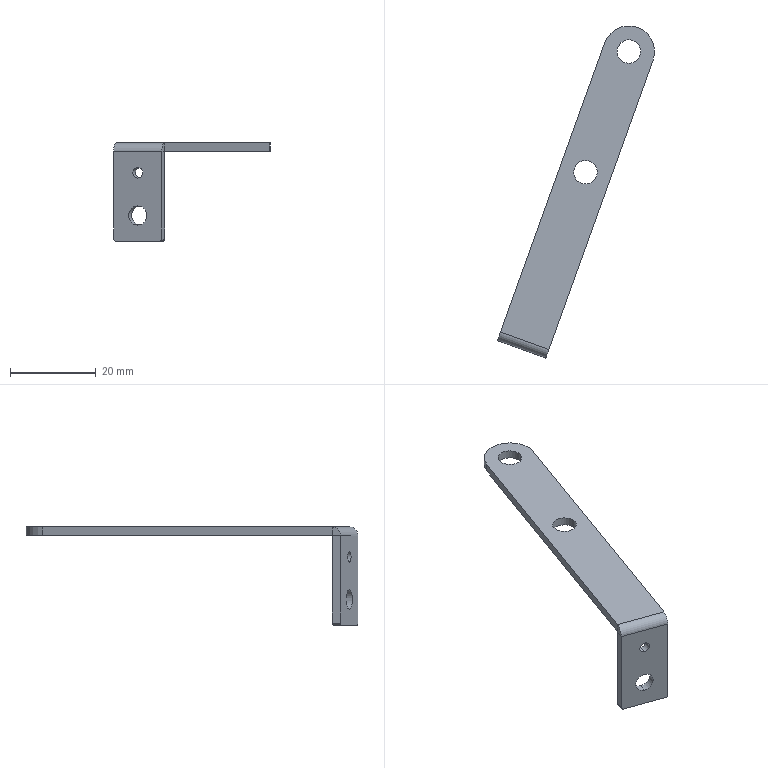Component | SolidWorks | CLS-MechanismAccessory4-1 | 1 solid | 25 faces | box 36.72 x 77.65 x 23 mm | volume 2245 mm3 | cylinder 14 | plane 11 | commonest cylinder face diameters 5.5 x4 2.5 x2 4.5 x2 12 x2 1 x2 4.2 x1 0.2 x1 | material 2.0 Galvanized Sheet Q235A
STEP:
#1=CARTESIAN_POINT('',(1.545,-2.454,-0.3445));
#2=VERTEX_POINT('',#1);
#3=CARTESIAN_POINT('',(1.545,-2.454,-0.4429));
#4=VERTEX_POINT('',#3);
#5=CARTESIAN_POINT('',(1.545,-2.454,-0.3937));
#6=DIRECTION('',(-0.3389,-0.9408,0.));
#7=DIRECTION('',(0.,-0.,-1.));
#8=AXIS2_PLACEMENT_3D('',#5,#6,#7);
#9=CIRCLE('',#8,0.04921);
#10=EDGE_CURVE('',#2,#4,#9,.T.);
#11=ORIENTED_EDGE('',*,*,#10,.F.);
#12=CARTESIAN_POINT('',(1.518,-2.528,-0.3445));
#13=VERTEX_POINT('',#12);
#14=CARTESIAN_POINT('',(1.545,-2.454,-0.3445));
#15=DIRECTION('',(-0.3389,-0.9408,0.));
#16=VECTOR('',#15,39.37);
#17=LINE('',#14,#16);
#18=EDGE_CURVE('',#2,#13,#17,.T.);
#19=ORIENTED_EDGE('',*,*,#18,.T.);
#20=CARTESIAN_POINT('',(1.518,-2.528,-0.4429));
#21=VERTEX_POINT('',#20);
#22=CARTESIAN_POINT('',(1.518,-2.528,-0.3937));
#23=DIRECTION('',(-0.3389,-0.9408,0.));
#24=DIRECTION('',(0.,0.,-1.));
#25=AXIS2_PLACEMENT_3D('',#22,#23,#24);
#26=CIRCLE('',#25,0.04921);
#27=EDGE_CURVE('',#13,#21,#26,.T.);
#28=ORIENTED_EDGE('',*,*,#27,.T.);
#29=CARTESIAN_POINT('',(1.545,-2.454,-0.4429));
#30=DIRECTION('',(-0.3389,-0.9408,0.));
#31=VECTOR('',#30,39.37);
#32=LINE('',#29,#31);
#33=EDGE_CURVE('',#4,#21,#32,.T.);
#34=ORIENTED_EDGE('',*,*,#33,.F.);
#35=EDGE_LOOP('',(#11,#19,#28,#34));
#36=FACE_OUTER_BOUND('',#35,.T.);
#37=CARTESIAN_POINT('',(1.545,-2.454,-0.3937));
#38=DIRECTION('',(-0.3389,-0.9408,0.));
#39=DIRECTION('',(0.,-0.,-1.));
#40=AXIS2_PLACEMENT_3D('',#37,#38,#39);
#41=CYLINDRICAL_SURFACE('',#40,0.04921);
#42=ADVANCED_FACE('',(#36),#41,.F.);
#43=CARTESIAN_POINT('',(1.545,-2.454,-0.6988));
#44=VERTEX_POINT('',#43);
#45=CARTESIAN_POINT('',(1.545,-2.454,-0.876));
#46=VERTEX_POINT('',#45);
#47=CARTESIAN_POINT('',(1.545,-2.454,-0.7874));
#48=DIRECTION('',(-0.3389,-0.9408,0.));
#49=DIRECTION('',(0.,-0.,-1.));
#50=AXIS2_PLACEMENT_3D('',#47,#48,#49);
#51=CIRCLE('',#50,0.08858);
#52=EDGE_CURVE('',#44,#46,#51,.T.);
#53=ORIENTED_EDGE('',*,*,#52,.F.);
#54=CARTESIAN_POINT('',(1.518,-2.528,-0.6988));
#55=VERTEX_POINT('',#54);
#56=CARTESIAN_POINT('',(1.545,-2.454,-0.6988));
#57=DIRECTION('',(-0.3389,-0.9408,0.));
#58=VECTOR('',#57,39.37);
#59=LINE('',#56,#58);
#60=EDGE_CURVE('',#44,#55,#59,.T.);
#61=ORIENTED_EDGE('',*,*,#60,.T.);
#62=CARTESIAN_POINT('',(1.518,-2.528,-0.876));
#63=VERTEX_POINT('',#62);
#64=CARTESIAN_POINT('',(1.518,-2.528,-0.7874));
#65=DIRECTION('',(-0.3389,-0.9408,0.));
#66=DIRECTION('',(0.,-0.,-1.));
#67=AXIS2_PLACEMENT_3D('',#64,#65,#66);
#68=CIRCLE('',#67,0.08858);
#69=EDGE_CURVE('',#55,#63,#68,.T.);
#70=ORIENTED_EDGE('',*,*,#69,.T.);
#71=CARTESIAN_POINT('',(1.545,-2.454,-0.876));
#72=DIRECTION('',(-0.3389,-0.9408,0.));
#73=VECTOR('',#72,39.37);
#74=LINE('',#71,#73);
#75=EDGE_CURVE('',#46,#63,#74,.T.);
#76=ORIENTED_EDGE('',*,*,#75,.F.);
#77=EDGE_LOOP('',(#53,#61,#70,#76));
#78=FACE_OUTER_BOUND('',#77,.T.);
#79=CARTESIAN_POINT('',(1.545,-2.454,-0.7874));
#80=DIRECTION('',(-0.3389,-0.9408,0.));
#81=DIRECTION('',(0.,-0.,-1.));
#82=AXIS2_PLACEMENT_3D('',#79,#80,#81);
#83=CYLINDRICAL_SURFACE('',#82,0.08858);
#84=ADVANCED_FACE('',(#78),#83,.F.);
#85=CARTESIAN_POINT('',(2.003,-0.8613,-0.1969));
#86=VERTEX_POINT('',#85);
#87=CARTESIAN_POINT('',(2.207,-0.9346,-0.1969));
#88=VERTEX_POINT('',#87);
#89=CARTESIAN_POINT('',(2.105,-0.8979,-0.1969));
#90=DIRECTION('',(0.,-0.,1.));
#91=DIRECTION('',(0.9408,-0.3389,0.));
#92=AXIS2_PLACEMENT_3D('',#89,#90,#91);
#93=CIRCLE('',#92,0.1083);
#94=EDGE_CURVE('',#86,#88,#93,.T.);
#95=ORIENTED_EDGE('',*,*,#94,.F.);
#96=CARTESIAN_POINT('',(2.003,-0.8613,-0.1181));
#97=VERTEX_POINT('',#96);
#98=CARTESIAN_POINT('',(2.003,-0.8613,-0.1969));
#99=DIRECTION('',(0.,-0.,1.));
#100=VECTOR('',#99,39.37);
#101=LINE('',#98,#100);
#102=EDGE_CURVE('',#86,#97,#101,.T.);
#103=ORIENTED_EDGE('',*,*,#102,.T.);
#104=CARTESIAN_POINT('',(2.207,-0.9346,-0.1181));
#105=VERTEX_POINT('',#104);
#106=CARTESIAN_POINT('',(2.105,-0.8979,-0.1181));
#107=DIRECTION('',(0.,-0.,1.));
#108=DIRECTION('',(0.9408,-0.3389,0.));
#109=AXIS2_PLACEMENT_3D('',#106,#107,#108);
#110=CIRCLE('',#109,0.1083);
#111=EDGE_CURVE('',#97,#105,#110,.T.);
#112=ORIENTED_EDGE('',*,*,#111,.T.);
#113=CARTESIAN_POINT('',(2.207,-0.9346,-0.1969));
#114=DIRECTION('',(0.,-0.,1.));
#115=VECTOR('',#114,39.37);
#116=LINE('',#113,#115);
#117=EDGE_CURVE('',#88,#105,#116,.T.);
#118=ORIENTED_EDGE('',*,*,#117,.F.);
#119=EDGE_LOOP('',(#95,#103,#112,#118));
#120=FACE_OUTER_BOUND('',#119,.T.);
#121=CARTESIAN_POINT('',(2.105,-0.8979,-0.1969));
#122=DIRECTION('',(0.,-0.,1.));
#123=DIRECTION('',(0.9408,-0.3389,0.));
#124=AXIS2_PLACEMENT_3D('',#121,#122,#123);
#125=CYLINDRICAL_SURFACE('',#124,0.1083);
#126=ADVANCED_FACE('',(#120),#125,.F.);
#127=CARTESIAN_POINT('',(2.404,0.25,-0.1969));
#128=VERTEX_POINT('',#127);
#129=CARTESIAN_POINT('',(2.607,0.1766,-0.1969));
#130=VERTEX_POINT('',#129);
#131=CARTESIAN_POINT('',(2.506,0.2133,-0.1969));
#132=DIRECTION('',(0.,-0.,1.));
#133=DIRECTION('',(0.9408,-0.3389,0.));
#134=AXIS2_PLACEMENT_3D('',#131,#132,#133);
#135=CIRCLE('',#134,0.1083);
#136=EDGE_CURVE('',#128,#130,#135,.T.);
#137=ORIENTED_EDGE('',*,*,#136,.F.);
#138=CARTESIAN_POINT('',(2.404,0.25,-0.1181));
#139=VERTEX_POINT('',#138);
#140=CARTESIAN_POINT('',(2.404,0.25,-0.1969));
#141=DIRECTION('',(0.,-0.,1.));
#142=VECTOR('',#141,39.37);
#143=LINE('',#140,#142);
#144=EDGE_CURVE('',#128,#139,#143,.T.);
#145=ORIENTED_EDGE('',*,*,#144,.T.);
#146=CARTESIAN_POINT('',(2.607,0.1766,-0.1181));
#147=VERTEX_POINT('',#146);
#148=CARTESIAN_POINT('',(2.506,0.2133,-0.1181));
#149=DIRECTION('',(0.,-0.,1.));
#150=DIRECTION('',(0.9408,-0.3389,0.));
#151=AXIS2_PLACEMENT_3D('',#148,#149,#150);
#152=CIRCLE('',#151,0.1083);
#153=EDGE_CURVE('',#139,#147,#152,.T.);
#154=ORIENTED_EDGE('',*,*,#153,.T.);
#155=CARTESIAN_POINT('',(2.607,0.1766,-0.1969));
#156=DIRECTION('',(0.,-0.,1.));
#157=VECTOR('',#156,39.37);
#158=LINE('',#155,#157);
#159=EDGE_CURVE('',#130,#147,#158,.T.);
#160=ORIENTED_EDGE('',*,*,#159,.F.);
#161=EDGE_LOOP('',(#137,#145,#154,#160));
#162=FACE_OUTER_BOUND('',#161,.T.);
#163=CARTESIAN_POINT('',(2.506,0.2133,-0.1969));
#164=DIRECTION('',(0.,-0.,1.));
#165=DIRECTION('',(0.9408,-0.3389,0.));
#166=AXIS2_PLACEMENT_3D('',#163,#164,#165);
#167=CYLINDRICAL_SURFACE('',#166,0.1083);
#168=ADVANCED_FACE('',(#162),#167,.F.);
#169=CARTESIAN_POINT('',(2.283,0.2933,-0.1969));
#170=VERTEX_POINT('',#169);
#171=CARTESIAN_POINT('',(1.324,-2.37,-0.1969));
#172=VERTEX_POINT('',#171);
#173=CARTESIAN_POINT('',(2.363,0.5156,-0.1969));
#174=DIRECTION('',(-0.3389,-0.9408,-0.));
#175=VECTOR('',#174,39.37);
#176=LINE('',#173,#175);
#177=EDGE_CURVE('',#170,#172,#176,.T.);
#178=ORIENTED_EDGE('',*,*,#177,.T.);
#179=CARTESIAN_POINT('',(1.324,-2.37,-0.1181));
#180=VERTEX_POINT('',#179);
#181=CARTESIAN_POINT('',(1.324,-2.37,-0.1969));
#182=DIRECTION('',(0.,-0.,1.));
#183=VECTOR('',#182,39.37);
#184=LINE('',#181,#183);
#185=EDGE_CURVE('',#172,#180,#184,.T.);
#186=ORIENTED_EDGE('',*,*,#185,.T.);
#187=CARTESIAN_POINT('',(2.283,0.2933,-0.1181));
#188=VERTEX_POINT('',#187);
#189=CARTESIAN_POINT('',(2.363,0.5156,-0.1181));
#190=DIRECTION('',(-0.3389,-0.9408,-0.));
#191=VECTOR('',#190,39.37);
#192=LINE('',#189,#191);
#193=EDGE_CURVE('',#188,#180,#192,.T.);
#194=ORIENTED_EDGE('',*,*,#193,.F.);
#195=CARTESIAN_POINT('',(2.283,0.2933,-0.1969));
#196=DIRECTION('',(-0.,0.,-1.));
#197=VECTOR('',#196,39.37);
#198=LINE('',#195,#197);
#199=EDGE_CURVE('',#188,#170,#198,.T.);
#200=ORIENTED_EDGE('',*,*,#199,.T.);
#201=EDGE_LOOP('',(#178,#186,#194,#200));
#202=FACE_OUTER_BOUND('',#201,.T.);
#203=CARTESIAN_POINT('',(2.363,0.5156,-0.1969));
#204=DIRECTION('',(-0.9408,0.3389,0.));
#205=DIRECTION('',(-0.3389,-0.9408,-0.));
#206=AXIS2_PLACEMENT_3D('',#203,#204,#205);
#207=PLANE('',#206);
#208=ADVANCED_FACE('',(#202),#207,.T.);
#209=CARTESIAN_POINT('',(2.105,-0.8979,-0.1969));
#210=DIRECTION('',(0.,-0.,1.));
#211=DIRECTION('',(0.9408,-0.3389,0.));
#212=AXIS2_PLACEMENT_3D('',#209,#210,#211);
#213=CIRCLE('',#212,0.1083);
#214=EDGE_CURVE('',#88,#86,#213,.T.);
#215=ORIENTED_EDGE('',*,*,#214,.T.);
#216=ORIENTED_EDGE('',*,*,#94,.T.);
#217=EDGE_LOOP('',(#215,#216));
#218=FACE_BOUND('',#217,.T.);
#219=CARTESIAN_POINT('',(2.506,0.2133,-0.1969));
#220=DIRECTION('',(0.,-0.,1.));
#221=DIRECTION('',(0.9408,-0.3389,0.));
#222=AXIS2_PLACEMENT_3D('',#219,#220,#221);
#223=CIRCLE('',#222,0.1083);
#224=EDGE_CURVE('',#130,#128,#223,.T.);
#225=ORIENTED_EDGE('',*,*,#224,.T.);
#226=ORIENTED_EDGE('',*,*,#136,.T.);
#227=EDGE_LOOP('',(#225,#226));
#228=FACE_BOUND('',#227,.T.);
#229=CARTESIAN_POINT('',(1.768,-2.53,-0.1969));
#230=VERTEX_POINT('',#229);
#231=CARTESIAN_POINT('',(2.728,0.1332,-0.1969));
#232=VERTEX_POINT('',#231);
#233=CARTESIAN_POINT('',(2.808,0.3555,-0.1969));
#234=DIRECTION('',(0.3389,0.9408,0.));
#235=VECTOR('',#234,39.37);
#236=LINE('',#233,#235);
#237=EDGE_CURVE('',#230,#232,#236,.T.);
#238=ORIENTED_EDGE('',*,*,#237,.F.);
#239=CARTESIAN_POINT('',(1.324,-2.37,-0.1969));
#240=DIRECTION('',(0.9408,-0.3389,-0.));
#241=VECTOR('',#240,39.37);
#242=LINE('',#239,#241);
#243=EDGE_CURVE('',#172,#230,#242,.T.);
#244=ORIENTED_EDGE('',*,*,#243,.F.);
#245=ORIENTED_EDGE('',*,*,#177,.F.);
#246=CARTESIAN_POINT('',(2.586,0.4355,-0.1969));
#247=VERTEX_POINT('',#246);
#248=CARTESIAN_POINT('',(2.506,0.2133,-0.1969));
#249=DIRECTION('',(-0.,0.,-1.));
#250=DIRECTION('',(-0.9408,0.3389,0.));
#251=AXIS2_PLACEMENT_3D('',#248,#249,#250);
#252=CIRCLE('',#251,0.2362);
#253=EDGE_CURVE('',#170,#247,#252,.T.);
#254=ORIENTED_EDGE('',*,*,#253,.T.);
#255=CARTESIAN_POINT('',(2.506,0.2133,-0.1969));
#256=DIRECTION('',(-0.,0.,-1.));
#257=DIRECTION('',(-0.9408,0.3389,0.));
#258=AXIS2_PLACEMENT_3D('',#255,#256,#257);
#259=CIRCLE('',#258,0.2362);
#260=EDGE_CURVE('',#247,#232,#259,.T.);
#261=ORIENTED_EDGE('',*,*,#260,.T.);
#262=EDGE_LOOP('',(#238,#244,#245,#254,#261));
#263=FACE_OUTER_BOUND('',#262,.T.);
#264=CARTESIAN_POINT('',(1.296,-2.448,-0.1969));
#265=DIRECTION('',(-0.,0.,-1.));
#266=DIRECTION('',(-0.9408,0.3389,0.));
#267=AXIS2_PLACEMENT_3D('',#264,#265,#266);
#268=PLANE('',#267);
#269=ADVANCED_FACE('',(#218,#228,#263),#268,.T.);
#270=CARTESIAN_POINT('',(2.506,0.2133,-0.1181));
#271=DIRECTION('',(0.,-0.,1.));
#272=DIRECTION('',(0.9408,-0.3389,0.));
#273=AXIS2_PLACEMENT_3D('',#270,#271,#272);
#274=CIRCLE('',#273,0.1083);
#275=EDGE_CURVE('',#147,#139,#274,.T.);
#276=ORIENTED_EDGE('',*,*,#275,.F.);
#277=ORIENTED_EDGE('',*,*,#153,.F.);
#278=EDGE_LOOP('',(#276,#277));
#279=FACE_BOUND('',#278,.T.);
#280=CARTESIAN_POINT('',(2.105,-0.8979,-0.1181));
#281=DIRECTION('',(0.,-0.,1.));
#282=DIRECTION('',(0.9408,-0.3389,0.));
#283=AXIS2_PLACEMENT_3D('',#280,#281,#282);
#284=CIRCLE('',#283,0.1083);
#285=EDGE_CURVE('',#105,#97,#284,.T.);
#286=ORIENTED_EDGE('',*,*,#285,.F.);
#287=ORIENTED_EDGE('',*,*,#111,.F.);
#288=EDGE_LOOP('',(#286,#287));
#289=FACE_BOUND('',#288,.T.);
#290=CARTESIAN_POINT('',(1.768,-2.53,-0.1181));
#291=VERTEX_POINT('',#290);
#292=CARTESIAN_POINT('',(1.324,-2.37,-0.1181));
#293=DIRECTION('',(0.9408,-0.3389,-0.));
#294=VECTOR('',#293,39.37);
#295=LINE('',#292,#294);
#296=EDGE_CURVE('',#180,#291,#295,.T.);
#297=ORIENTED_EDGE('',*,*,#296,.T.);
#298=CARTESIAN_POINT('',(2.728,0.1332,-0.1181));
#299=VERTEX_POINT('',#298);
#300=CARTESIAN_POINT('',(2.808,0.3555,-0.1181));
#301=DIRECTION('',(0.3389,0.9408,0.));
#302=VECTOR('',#301,39.37);
#303=LINE('',#300,#302);
#304=EDGE_CURVE('',#291,#299,#303,.T.);
#305=ORIENTED_EDGE('',*,*,#304,.T.);
#306=CARTESIAN_POINT('',(2.586,0.4355,-0.1181));
#307=VERTEX_POINT('',#306);
#308=CARTESIAN_POINT('',(2.506,0.2133,-0.1181));
#309=DIRECTION('',(0.,-0.,1.));
#310=DIRECTION('',(-0.9408,0.3389,0.));
#311=AXIS2_PLACEMENT_3D('',#308,#309,#310);
#312=CIRCLE('',#311,0.2362);
#313=EDGE_CURVE('',#299,#307,#312,.T.);
#314=ORIENTED_EDGE('',*,*,#313,.T.);
#315=CARTESIAN_POINT('',(2.506,0.2133,-0.1181));
#316=DIRECTION('',(0.,-0.,1.));
#317=DIRECTION('',(-0.9408,0.3389,0.));
#318=AXIS2_PLACEMENT_3D('',#315,#316,#317);
#319=CIRCLE('',#318,0.2362);
#320=EDGE_CURVE('',#307,#188,#319,.T.);
#321=ORIENTED_EDGE('',*,*,#320,.T.);
#322=ORIENTED_EDGE('',*,*,#193,.T.);
#323=EDGE_LOOP('',(#297,#305,#314,#321,#322));
#324=FACE_OUTER_BOUND('',#323,.T.);
#325=CARTESIAN_POINT('',(1.296,-2.448,-0.1181));
#326=DIRECTION('',(-0.,0.,-1.));
#327=DIRECTION('',(-0.9408,0.3389,0.));
#328=AXIS2_PLACEMENT_3D('',#325,#326,#327);
#329=PLANE('',#328);
#330=ADVANCED_FACE('',(#279,#289,#324),#329,.F.);
#331=CARTESIAN_POINT('',(1.768,-2.53,-0.1969));
#332=DIRECTION('',(0.,-0.,1.));
#333=VECTOR('',#332,39.37);
#334=LINE('',#331,#333);
#335=EDGE_CURVE('',#230,#291,#334,.T.);
#336=ORIENTED_EDGE('',*,*,#335,.F.);
#337=ORIENTED_EDGE('',*,*,#237,.T.);
#338=CARTESIAN_POINT('',(2.728,0.1332,-0.1969));
#339=DIRECTION('',(0.,-0.,1.));
#340=VECTOR('',#339,39.37);
#341=LINE('',#338,#340);
#342=EDGE_CURVE('',#232,#299,#341,.T.);
#343=ORIENTED_EDGE('',*,*,#342,.T.);
#344=ORIENTED_EDGE('',*,*,#304,.F.);
#345=EDGE_LOOP('',(#336,#337,#343,#344));
#346=FACE_OUTER_BOUND('',#345,.T.);
#347=CARTESIAN_POINT('',(2.808,0.3555,-0.1969));
#348=DIRECTION('',(0.9408,-0.3389,-0.));
#349=DIRECTION('',(0.3389,0.9408,0.));
#350=AXIS2_PLACEMENT_3D('',#347,#348,#349);
#351=PLANE('',#350);
#352=ADVANCED_FACE('',(#346),#351,.T.);
#353=ORIENTED_EDGE('',*,*,#144,.F.);
#354=ORIENTED_EDGE('',*,*,#224,.F.);
#355=ORIENTED_EDGE('',*,*,#159,.T.);
#356=ORIENTED_EDGE('',*,*,#275,.T.);
#357=EDGE_LOOP('',(#353,#354,#355,#356));
#358=FACE_OUTER_BOUND('',#357,.T.);
#359=CARTESIAN_POINT('',(2.506,0.2133,-0.1969));
#360=DIRECTION('',(0.,-0.,1.));
#361=DIRECTION('',(0.9408,-0.3389,0.));
#362=AXIS2_PLACEMENT_3D('',#359,#360,#361);
#363=CYLINDRICAL_SURFACE('',#362,0.1083);
#364=ADVANCED_FACE('',(#358),#363,.F.);
#365=ORIENTED_EDGE('',*,*,#102,.F.);
#366=ORIENTED_EDGE('',*,*,#214,.F.);
#367=ORIENTED_EDGE('',*,*,#117,.T.);
#368=ORIENTED_EDGE('',*,*,#285,.T.);
#369=EDGE_LOOP('',(#365,#366,#367,#368));
#370=FACE_OUTER_BOUND('',#369,.T.);
#371=CARTESIAN_POINT('',(2.105,-0.8979,-0.1969));
#372=DIRECTION('',(0.,-0.,1.));
#373=DIRECTION('',(0.9408,-0.3389,0.));
#374=AXIS2_PLACEMENT_3D('',#371,#372,#373);
#375=CYLINDRICAL_SURFACE('',#374,0.1083);
#376=ADVANCED_FACE('',(#370),#375,.F.);
#377=ORIENTED_EDGE('',*,*,#342,.F.);
#378=ORIENTED_EDGE('',*,*,#260,.F.);
#379=CARTESIAN_POINT('',(2.586,0.4355,-0.1969));
#380=DIRECTION('',(-0.,0.,-1.));
#381=VECTOR('',#380,39.37);
#382=LINE('',#379,#381);
#383=EDGE_CURVE('',#307,#247,#382,.T.);
#384=ORIENTED_EDGE('',*,*,#383,.F.);
#385=ORIENTED_EDGE('',*,*,#313,.F.);
#386=EDGE_LOOP('',(#377,#378,#384,#385));
#387=FACE_OUTER_BOUND('',#386,.T.);
#388=CARTESIAN_POINT('',(2.506,0.2133,-0.1969));
#389=DIRECTION('',(0.,-0.,1.));
#390=DIRECTION('',(0.9408,-0.3389,0.));
#391=AXIS2_PLACEMENT_3D('',#388,#389,#390);
#392=CYLINDRICAL_SURFACE('',#391,0.2362);
#393=ADVANCED_FACE('',(#387),#392,.T.);
#394=ORIENTED_EDGE('',*,*,#253,.F.);
#395=ORIENTED_EDGE('',*,*,#199,.F.);
#396=ORIENTED_EDGE('',*,*,#320,.F.);
#397=ORIENTED_EDGE('',*,*,#383,.T.);
#398=EDGE_LOOP('',(#394,#395,#396,#397));
#399=FACE_OUTER_BOUND('',#398,.T.);
#400=CARTESIAN_POINT('',(2.506,0.2133,-0.1969));
#401=DIRECTION('',(0.,-0.,1.));
#402=DIRECTION('',(0.9408,-0.3389,0.));
#403=AXIS2_PLACEMENT_3D('',#400,#401,#402);
#404=CYLINDRICAL_SURFACE('',#403,0.2362);
#405=ADVANCED_FACE('',(#399),#404,.T.);
#406=CARTESIAN_POINT('',(1.767,-2.534,-0.2008));
#407=VERTEX_POINT('',#406);
#408=CARTESIAN_POINT('',(1.74,-2.608,-0.2008));
#409=VERTEX_POINT('',#408);
#410=CARTESIAN_POINT('',(1.74,-2.608,-0.2008));
#411=DIRECTION('',(-0.3389,-0.9408,0.));
#412=VECTOR('',#411,39.37);
#413=LINE('',#410,#412);
#414=EDGE_CURVE('',#407,#409,#413,.T.);
#415=ORIENTED_EDGE('',*,*,#414,.F.);
#416=CARTESIAN_POINT('',(1.768,-2.53,-0.2008));
#417=DIRECTION('',(0.9408,-0.3389,-0.));
#418=DIRECTION('',(0.,0.,1.));
#419=AXIS2_PLACEMENT_3D('',#416,#417,#418);
#420=CIRCLE('',#419,0.003937);
#421=EDGE_CURVE('',#230,#407,#420,.T.);
#422=ORIENTED_EDGE('',*,*,#421,.F.);
#423=ORIENTED_EDGE('',*,*,#335,.T.);
#424=CARTESIAN_POINT('',(1.768,-2.53,-0.2008));
#425=DIRECTION('',(0.9408,-0.3389,-0.));
#426=DIRECTION('',(0.,0.,1.));
#427=AXIS2_PLACEMENT_3D('',#424,#425,#426);
#428=CIRCLE('',#427,0.08268);
#429=EDGE_CURVE('',#291,#409,#428,.T.);
#430=ORIENTED_EDGE('',*,*,#429,.T.);
#431=EDGE_LOOP('',(#415,#422,#423,#430));
#432=FACE_OUTER_BOUND('',#431,.T.);
#433=CARTESIAN_POINT('',(1.768,-2.53,-0.2008));
#434=DIRECTION('',(0.9408,-0.3389,-0.));
#435=DIRECTION('',(-0.,0.,-1.));
#436=AXIS2_PLACEMENT_3D('',#433,#434,#435);
#437=PLANE('',#436);
#438=ADVANCED_FACE('',(#432),#437,.T.);
#439=CARTESIAN_POINT('',(1.323,-2.374,-0.2008));
#440=VERTEX_POINT('',#439);
#441=CARTESIAN_POINT('',(1.324,-2.37,-0.2008));
#442=DIRECTION('',(-0.9408,0.3389,0.));
#443=DIRECTION('',(0.,0.,1.));
#444=AXIS2_PLACEMENT_3D('',#441,#442,#443);
#445=CIRCLE('',#444,0.003937);
#446=EDGE_CURVE('',#440,#172,#445,.T.);
#447=ORIENTED_EDGE('',*,*,#446,.F.);
#448=CARTESIAN_POINT('',(1.296,-2.448,-0.2008));
#449=VERTEX_POINT('',#448);
#450=CARTESIAN_POINT('',(1.323,-2.374,-0.2008));
#451=DIRECTION('',(-0.3389,-0.9408,0.));
#452=VECTOR('',#451,39.37);
#453=LINE('',#450,#452);
#454=EDGE_CURVE('',#440,#449,#453,.T.);
#455=ORIENTED_EDGE('',*,*,#454,.T.);
#456=CARTESIAN_POINT('',(1.324,-2.37,-0.2008));
#457=DIRECTION('',(-0.9408,0.3389,0.));
#458=DIRECTION('',(0.,0.,1.));
#459=AXIS2_PLACEMENT_3D('',#456,#457,#458);
#460=CIRCLE('',#459,0.08268);
#461=EDGE_CURVE('',#449,#180,#460,.T.);
#462=ORIENTED_EDGE('',*,*,#461,.T.);
#463=ORIENTED_EDGE('',*,*,#185,.F.);
#464=EDGE_LOOP('',(#447,#455,#462,#463));
#465=FACE_OUTER_BOUND('',#464,.T.);
#466=CARTESIAN_POINT('',(1.324,-2.37,-0.2008));
#467=DIRECTION('',(0.9408,-0.3389,-0.));
#468=DIRECTION('',(-0.,0.,-1.));
#469=AXIS2_PLACEMENT_3D('',#466,#467,#468);
#470=PLANE('',#469);
#471=ADVANCED_FACE('',(#465),#470,.F.);
#472=ORIENTED_EDGE('',*,*,#296,.F.);
#473=ORIENTED_EDGE('',*,*,#461,.F.);
#474=CARTESIAN_POINT('',(1.74,-2.608,-0.2008));
#475=DIRECTION('',(0.9408,-0.3389,-0.));
#476=VECTOR('',#475,39.37);
#477=LINE('',#474,#476);
#478=EDGE_CURVE('',#449,#409,#477,.T.);
#479=ORIENTED_EDGE('',*,*,#478,.T.);
#480=ORIENTED_EDGE('',*,*,#429,.F.);
#481=EDGE_LOOP('',(#472,#473,#479,#480));
#482=FACE_OUTER_BOUND('',#481,.T.);
#483=CARTESIAN_POINT('',(1.324,-2.37,-0.2008));
#484=DIRECTION('',(-0.9408,0.3389,0.));
#485=DIRECTION('',(-0.3389,-0.9408,0.));
#486=AXIS2_PLACEMENT_3D('',#483,#484,#485);
#487=CYLINDRICAL_SURFACE('',#486,0.08268);
#488=ADVANCED_FACE('',(#482),#487,.T.);
#489=ORIENTED_EDGE('',*,*,#243,.T.);
#490=ORIENTED_EDGE('',*,*,#421,.T.);
#491=CARTESIAN_POINT('',(1.767,-2.534,-0.2008));
#492=DIRECTION('',(-0.9408,0.3389,0.));
#493=VECTOR('',#492,39.37);
#494=LINE('',#491,#493);
#495=EDGE_CURVE('',#407,#440,#494,.T.);
#496=ORIENTED_EDGE('',*,*,#495,.T.);
#497=ORIENTED_EDGE('',*,*,#446,.T.);
#498=EDGE_LOOP('',(#489,#490,#496,#497));
#499=FACE_OUTER_BOUND('',#498,.T.);
#500=CARTESIAN_POINT('',(1.324,-2.37,-0.2008));
#501=DIRECTION('',(-0.9408,0.3389,0.));
#502=DIRECTION('',(-0.3389,-0.9408,0.));
#503=AXIS2_PLACEMENT_3D('',#500,#501,#502);
#504=CYLINDRICAL_SURFACE('',#503,0.003937);
#505=ADVANCED_FACE('',(#499),#504,.F.);
#506=CARTESIAN_POINT('',(1.323,-2.374,-1.004));
#507=VERTEX_POINT('',#506);
#508=CARTESIAN_POINT('',(1.323,-2.374,-1.024));
#509=DIRECTION('',(-0.,-0.,-1.));
#510=VECTOR('',#509,39.37);
#511=LINE('',#508,#510);
#512=EDGE_CURVE('',#440,#507,#511,.T.);
#513=ORIENTED_EDGE('',*,*,#512,.T.);
#514=CARTESIAN_POINT('',(1.296,-2.448,-1.004));
#515=VERTEX_POINT('',#514);
#516=CARTESIAN_POINT('',(1.296,-2.448,-1.004));
#517=DIRECTION('',(-0.3389,-0.9408,0.));
#518=VECTOR('',#517,39.37);
#519=LINE('',#516,#518);
#520=EDGE_CURVE('',#507,#515,#519,.T.);
#521=ORIENTED_EDGE('',*,*,#520,.T.);
#522=CARTESIAN_POINT('',(1.296,-2.448,-0.1969));
#523=DIRECTION('',(-0.,-0.,-1.));
#524=VECTOR('',#523,39.37);
#525=LINE('',#522,#524);
#526=EDGE_CURVE('',#449,#515,#525,.T.);
#527=ORIENTED_EDGE('',*,*,#526,.F.);
#528=ORIENTED_EDGE('',*,*,#454,.F.);
#529=EDGE_LOOP('',(#513,#521,#527,#528));
#530=FACE_OUTER_BOUND('',#529,.T.);
#531=CARTESIAN_POINT('',(1.296,-2.448,-1.024));
#532=DIRECTION('',(0.9408,-0.3389,-0.));
#533=DIRECTION('',(0.3389,0.9408,0.));
#534=AXIS2_PLACEMENT_3D('',#531,#532,#533);
#535=PLANE('',#534);
#536=ADVANCED_FACE('',(#530),#535,.F.);
#537=CARTESIAN_POINT('',(1.74,-2.608,-1.004));
#538=VERTEX_POINT('',#537);
#539=CARTESIAN_POINT('',(1.74,-2.608,-0.1969));
#540=DIRECTION('',(0.,0.,1.));
#541=VECTOR('',#540,39.37);
#542=LINE('',#539,#541);
#543=EDGE_CURVE('',#538,#409,#542,.T.);
#544=ORIENTED_EDGE('',*,*,#543,.F.);
#545=CARTESIAN_POINT('',(1.767,-2.534,-1.004));
#546=VERTEX_POINT('',#545);
#547=CARTESIAN_POINT('',(1.74,-2.608,-1.004));
#548=DIRECTION('',(0.3389,0.9408,-0.));
#549=VECTOR('',#548,39.37);
#550=LINE('',#547,#549);
#551=EDGE_CURVE('',#538,#546,#550,.T.);
#552=ORIENTED_EDGE('',*,*,#551,.T.);
#553=CARTESIAN_POINT('',(1.767,-2.534,-0.1969));
#554=DIRECTION('',(0.,0.,1.));
#555=VECTOR('',#554,39.37);
#556=LINE('',#553,#555);
#557=EDGE_CURVE('',#546,#407,#556,.T.);
#558=ORIENTED_EDGE('',*,*,#557,.T.);
#559=ORIENTED_EDGE('',*,*,#414,.T.);
#560=EDGE_LOOP('',(#544,#552,#558,#559));
#561=FACE_OUTER_BOUND('',#560,.T.);
#562=CARTESIAN_POINT('',(1.74,-2.608,-0.1969));
#563=DIRECTION('',(-0.9408,0.3389,0.));
#564=DIRECTION('',(-0.3389,-0.9408,-0.));
#565=AXIS2_PLACEMENT_3D('',#562,#563,#564);
#566=PLANE('',#565);
#567=ADVANCED_FACE('',(#561),#566,.F.);
#568=CARTESIAN_POINT('',(1.518,-2.528,-0.3937));
#569=DIRECTION('',(-0.3389,-0.9408,0.));
#570=DIRECTION('',(0.,0.,-1.));
#571=AXIS2_PLACEMENT_3D('',#568,#569,#570);
#572=CIRCLE('',#571,0.04921);
#573=EDGE_CURVE('',#21,#13,#572,.T.);
#574=ORIENTED_EDGE('',*,*,#573,.F.);
#575=ORIENTED_EDGE('',*,*,#27,.F.);
#576=EDGE_LOOP('',(#574,#575));
#577=FACE_BOUND('',#576,.T.);
#578=CARTESIAN_POINT('',(1.518,-2.528,-0.7874));
#579=DIRECTION('',(-0.3389,-0.9408,0.));
#580=DIRECTION('',(0.,-0.,-1.));
#581=AXIS2_PLACEMENT_3D('',#578,#579,#580);
#582=CIRCLE('',#581,0.08858);
#583=EDGE_CURVE('',#63,#55,#582,.T.);
#584=ORIENTED_EDGE('',*,*,#583,.F.);
#585=ORIENTED_EDGE('',*,*,#69,.F.);
#586=EDGE_LOOP('',(#584,#585));
#587=FACE_BOUND('',#586,.T.);
#588=CARTESIAN_POINT('',(1.314,-2.454,-1.024));
#589=VERTEX_POINT('',#588);
#590=CARTESIAN_POINT('',(1.722,-2.601,-1.024));
#591=VERTEX_POINT('',#590);
#592=CARTESIAN_POINT('',(1.296,-2.448,-1.024));
#593=DIRECTION('',(0.9408,-0.3389,-0.));
#594=VECTOR('',#593,39.37);
#595=LINE('',#592,#594);
#596=EDGE_CURVE('',#589,#591,#595,.T.);
#597=ORIENTED_EDGE('',*,*,#596,.T.);
#598=CARTESIAN_POINT('',(1.722,-2.601,-1.004));
#599=DIRECTION('',(-0.3389,-0.9408,0.));
#600=DIRECTION('',(0.,0.,1.));
#601=AXIS2_PLACEMENT_3D('',#598,#599,#600);
#602=CIRCLE('',#601,0.01969);
#603=EDGE_CURVE('',#591,#538,#602,.T.);
#604=ORIENTED_EDGE('',*,*,#603,.T.);
#605=ORIENTED_EDGE('',*,*,#543,.T.);
#606=ORIENTED_EDGE('',*,*,#478,.F.);
#607=ORIENTED_EDGE('',*,*,#526,.T.);
#608=CARTESIAN_POINT('',(1.314,-2.454,-1.004));
#609=DIRECTION('',(-0.3389,-0.9408,0.));
#610=DIRECTION('',(0.,0.,1.));
#611=AXIS2_PLACEMENT_3D('',#608,#609,#610);
#612=CIRCLE('',#611,0.01969);
#613=EDGE_CURVE('',#515,#589,#612,.T.);
#614=ORIENTED_EDGE('',*,*,#613,.T.);
#615=EDGE_LOOP('',(#597,#604,#605,#606,#607,#614));
#616=FACE_OUTER_BOUND('',#615,.T.);
#617=CARTESIAN_POINT('',(1.296,-2.448,-0.1969));
#618=DIRECTION('',(0.3389,0.9408,-0.));
#619=DIRECTION('',(0.,0.,1.));
#620=AXIS2_PLACEMENT_3D('',#617,#618,#619);
#621=PLANE('',#620);
#622=ADVANCED_FACE('',(#577,#587,#616),#621,.F.);
#623=CARTESIAN_POINT('',(1.545,-2.454,-0.3937));
#624=DIRECTION('',(-0.3389,-0.9408,0.));
#625=DIRECTION('',(0.,-0.,-1.));
#626=AXIS2_PLACEMENT_3D('',#623,#624,#625);
#627=CIRCLE('',#626,0.04921);
#628=EDGE_CURVE('',#4,#2,#627,.T.);
#629=ORIENTED_EDGE('',*,*,#628,.T.);
#630=ORIENTED_EDGE('',*,*,#10,.T.);
#631=EDGE_LOOP('',(#629,#630));
#632=FACE_BOUND('',#631,.T.);
#633=CARTESIAN_POINT('',(1.545,-2.454,-0.7874));
#634=DIRECTION('',(-0.3389,-0.9408,0.));
#635=DIRECTION('',(0.,-0.,-1.));
#636=AXIS2_PLACEMENT_3D('',#633,#634,#635);
#637=CIRCLE('',#636,0.08858);
#638=EDGE_CURVE('',#46,#44,#637,.T.);
#639=ORIENTED_EDGE('',*,*,#638,.T.);
#640=ORIENTED_EDGE('',*,*,#52,.T.);
#641=EDGE_LOOP('',(#639,#640));
#642=FACE_BOUND('',#641,.T.);
#643=ORIENTED_EDGE('',*,*,#557,.F.);
#644=CARTESIAN_POINT('',(1.749,-2.527,-1.024));
#645=VERTEX_POINT('',#644);
#646=CARTESIAN_POINT('',(1.749,-2.527,-1.004));
#647=DIRECTION('',(0.3389,0.9408,-0.));
#648=DIRECTION('',(0.,0.,1.));
#649=AXIS2_PLACEMENT_3D('',#646,#647,#648);
#650=CIRCLE('',#649,0.01969);
#651=EDGE_CURVE('',#546,#645,#650,.T.);
#652=ORIENTED_EDGE('',*,*,#651,.T.);
#653=CARTESIAN_POINT('',(1.341,-2.38,-1.024));
#654=VERTEX_POINT('',#653);
#655=CARTESIAN_POINT('',(1.767,-2.534,-1.024));
#656=DIRECTION('',(0.9408,-0.3389,-0.));
#657=VECTOR('',#656,39.37);
#658=LINE('',#655,#657);
#659=EDGE_CURVE('',#654,#645,#658,.T.);
#660=ORIENTED_EDGE('',*,*,#659,.F.);
#661=CARTESIAN_POINT('',(1.341,-2.38,-1.004));
#662=DIRECTION('',(0.3389,0.9408,-0.));
#663=DIRECTION('',(0.,0.,1.));
#664=AXIS2_PLACEMENT_3D('',#661,#662,#663);
#665=CIRCLE('',#664,0.01969);
#666=EDGE_CURVE('',#654,#507,#665,.T.);
#667=ORIENTED_EDGE('',*,*,#666,.T.);
#668=ORIENTED_EDGE('',*,*,#512,.F.);
#669=ORIENTED_EDGE('',*,*,#495,.F.);
#670=EDGE_LOOP('',(#643,#652,#660,#667,#668,#669));
#671=FACE_OUTER_BOUND('',#670,.T.);
#672=CARTESIAN_POINT('',(1.323,-2.374,-0.1969));
#673=DIRECTION('',(0.3389,0.9408,-0.));
#674=DIRECTION('',(0.,0.,1.));
#675=AXIS2_PLACEMENT_3D('',#672,#673,#674);
#676=PLANE('',#675);
#677=ADVANCED_FACE('',(#632,#642,#671),#676,.T.);
#678=ORIENTED_EDGE('',*,*,#659,.T.);
#679=CARTESIAN_POINT('',(1.722,-2.601,-1.024));
#680=DIRECTION('',(-0.3389,-0.9408,0.));
#681=VECTOR('',#680,39.37);
#682=LINE('',#679,#681);
#683=EDGE_CURVE('',#645,#591,#682,.T.);
#684=ORIENTED_EDGE('',*,*,#683,.T.);
#685=ORIENTED_EDGE('',*,*,#596,.F.);
#686=CARTESIAN_POINT('',(1.314,-2.454,-1.024));
#687=DIRECTION('',(0.3389,0.9408,-0.));
#688=VECTOR('',#687,39.37);
#689=LINE('',#686,#688);
#690=EDGE_CURVE('',#589,#654,#689,.T.);
#691=ORIENTED_EDGE('',*,*,#690,.T.);
#692=EDGE_LOOP('',(#678,#684,#685,#691));
#693=FACE_OUTER_BOUND('',#692,.T.);
#694=CARTESIAN_POINT('',(1.74,-2.608,-1.024));
#695=DIRECTION('',(0.,0.,1.));
#696=DIRECTION('',(-0.3389,-0.9408,0.));
#697=AXIS2_PLACEMENT_3D('',#694,#695,#696);
#698=PLANE('',#697);
#699=ADVANCED_FACE('',(#693),#698,.F.);
#700=ORIENTED_EDGE('',*,*,#60,.F.);
#701=ORIENTED_EDGE('',*,*,#638,.F.);
#702=ORIENTED_EDGE('',*,*,#75,.T.);
#703=ORIENTED_EDGE('',*,*,#583,.T.);
#704=EDGE_LOOP('',(#700,#701,#702,#703));
#705=FACE_OUTER_BOUND('',#704,.T.);
#706=CARTESIAN_POINT('',(1.545,-2.454,-0.7874));
#707=DIRECTION('',(-0.3389,-0.9408,0.));
#708=DIRECTION('',(0.,-0.,-1.));
#709=AXIS2_PLACEMENT_3D('',#706,#707,#708);
#710=CYLINDRICAL_SURFACE('',#709,0.08858);
#711=ADVANCED_FACE('',(#705),#710,.F.);
#712=ORIENTED_EDGE('',*,*,#18,.F.);
#713=ORIENTED_EDGE('',*,*,#628,.F.);
#714=ORIENTED_EDGE('',*,*,#33,.T.);
#715=ORIENTED_EDGE('',*,*,#573,.T.);
#716=EDGE_LOOP('',(#712,#713,#714,#715));
#717=FACE_OUTER_BOUND('',#716,.T.);
#718=CARTESIAN_POINT('',(1.545,-2.454,-0.3937));
#719=DIRECTION('',(-0.3389,-0.9408,0.));
#720=DIRECTION('',(0.,-0.,-1.));
#721=AXIS2_PLACEMENT_3D('',#718,#719,#720);
#722=CYLINDRICAL_SURFACE('',#721,0.04921);
#723=ADVANCED_FACE('',(#717),#722,.F.);
#724=ORIENTED_EDGE('',*,*,#603,.F.);
#725=ORIENTED_EDGE('',*,*,#683,.F.);
#726=ORIENTED_EDGE('',*,*,#651,.F.);
#727=ORIENTED_EDGE('',*,*,#551,.F.);
#728=EDGE_LOOP('',(#724,#725,#726,#727));
#729=FACE_OUTER_BOUND('',#728,.T.);
#730=CARTESIAN_POINT('',(1.722,-2.601,-1.004));
#731=DIRECTION('',(0.3389,0.9408,-0.));
#732=DIRECTION('',(0.,0.,1.));
#733=AXIS2_PLACEMENT_3D('',#730,#731,#732);
#734=CYLINDRICAL_SURFACE('',#733,0.01969);
#735=ADVANCED_FACE('',(#729),#734,.T.);
#736=ORIENTED_EDGE('',*,*,#613,.F.);
#737=ORIENTED_EDGE('',*,*,#520,.F.);
#738=ORIENTED_EDGE('',*,*,#666,.F.);
#739=ORIENTED_EDGE('',*,*,#690,.F.);
#740=EDGE_LOOP('',(#736,#737,#738,#739));
#741=FACE_OUTER_BOUND('',#740,.T.);
#742=CARTESIAN_POINT('',(1.314,-2.454,-1.004));
#743=DIRECTION('',(0.3389,0.9408,-0.));
#744=DIRECTION('',(0.,0.,1.));
#745=AXIS2_PLACEMENT_3D('',#742,#743,#744);
#746=CYLINDRICAL_SURFACE('',#745,0.01969);
#747=ADVANCED_FACE('',(#741),#746,.T.);
#748=CLOSED_SHELL('',(#42,#84,#126,#168,#208,#269,#330,#352,#364,#376,#393,#405,#438,#471,#488,#505,#536,#567,#622,#677,#699,#711,#723,#735,#747));
#749=MANIFOLD_SOLID_BREP('',#748);
#750=CARTESIAN_POINT('',(0.,0.,0.));
#751=DIRECTION('',(0.,0.,1.));
#752=DIRECTION('',(1.,0.,0.));
#753=AXIS2_PLACEMENT_3D('',#750,#751,#752);
#754=(LENGTH_UNIT()NAMED_UNIT(*)SI_UNIT($,.METRE.));
#755=LENGTH_MEASURE_WITH_UNIT(LENGTH_MEASURE(0.0254),#754);
#756=DIMENSIONAL_EXPONENTS(1.,0.,0.,0.,0.,0.,0.);
#757=(CONVERSION_BASED_UNIT('',#755)LENGTH_UNIT()NAMED_UNIT(#756));
#758=UNCERTAINTY_MEASURE_WITH_UNIT(LENGTH_MEASURE(0.00001),#757,'','');
#759=(NAMED_UNIT(*)PLANE_ANGLE_UNIT()SI_UNIT($,.RADIAN.));
#760=(NAMED_UNIT(*)SI_UNIT($,.STERADIAN.)SOLID_ANGLE_UNIT());
#761=(GEOMETRIC_REPRESENTATION_CONTEXT(3)GLOBAL_UNCERTAINTY_ASSIGNED_CONTEXT((#758))GLOBAL_UNIT_ASSIGNED_CONTEXT((#757,#759,#760))REPRESENTATION_CONTEXT('',''));
#762=ADVANCED_BREP_SHAPE_REPRESENTATION('',(#749,#753),#761);
#763=COLOUR_RGB('',0.7922,0.8196,0.9333);
#764=FILL_AREA_STYLE_COLOUR('',#763);
#765=FILL_AREA_STYLE('',(#764));
#766=SURFACE_STYLE_FILL_AREA(#765);
#767=SURFACE_SIDE_STYLE('',(#766));
#768=SURFACE_STYLE_USAGE(.BOTH.,#767);
#769=PRESENTATION_STYLE_ASSIGNMENT((#768));
#770=STYLED_ITEM('',(#769),#749);
#771=PRESENTATION_LAYER_ASSIGNMENT('','',(#770));
#772=(LENGTH_UNIT()NAMED_UNIT(*)SI_UNIT($,.METRE.));
#773=LENGTH_MEASURE_WITH_UNIT(LENGTH_MEASURE(0.0254),#772);
#774=DIMENSIONAL_EXPONENTS(1.,0.,0.,0.,0.,0.,0.);
#775=(CONVERSION_BASED_UNIT('',#773)LENGTH_UNIT()NAMED_UNIT(#774));
#776=UNCERTAINTY_MEASURE_WITH_UNIT(LENGTH_MEASURE(0.00001),#775,'','');
#777=(NAMED_UNIT(*)PLANE_ANGLE_UNIT()SI_UNIT($,.RADIAN.));
#778=(NAMED_UNIT(*)SI_UNIT($,.STERADIAN.)SOLID_ANGLE_UNIT());
#779=(GEOMETRIC_REPRESENTATION_CONTEXT(3)GLOBAL_UNCERTAINTY_ASSIGNED_CONTEXT((#776))GLOBAL_UNIT_ASSIGNED_CONTEXT((#775,#777,#778))REPRESENTATION_CONTEXT('',''));
#780=MECHANICAL_DESIGN_GEOMETRIC_PRESENTATION_REPRESENTATION('',(#770),#779);